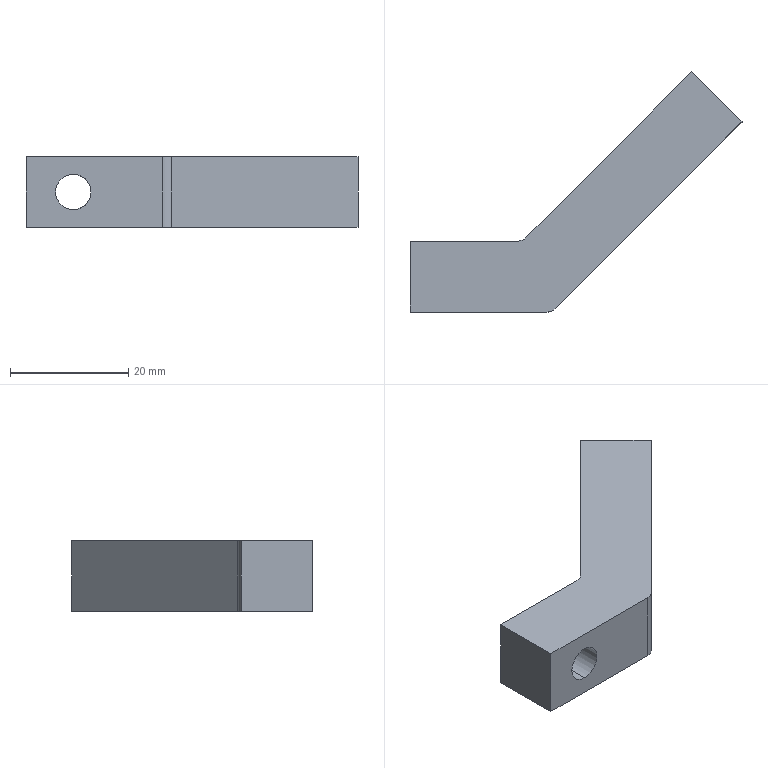CAM job | Mastercam | mm | 14 operations | part box 56.17 x 40.66 x 12
1. Facing | 24 - 100 平铣刀
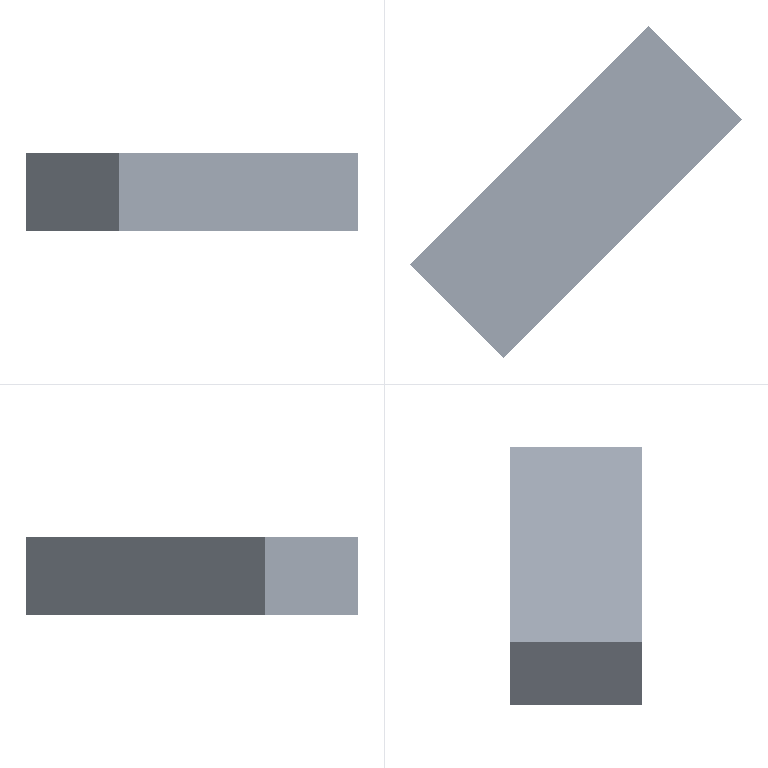2. Contour (Ramp) | 10 - 10 平铣刀
3. Surface Finish Flowline | 11 - 10 圆鼻铣刀
4. Contour (2D) | 10 - 10 平铣刀
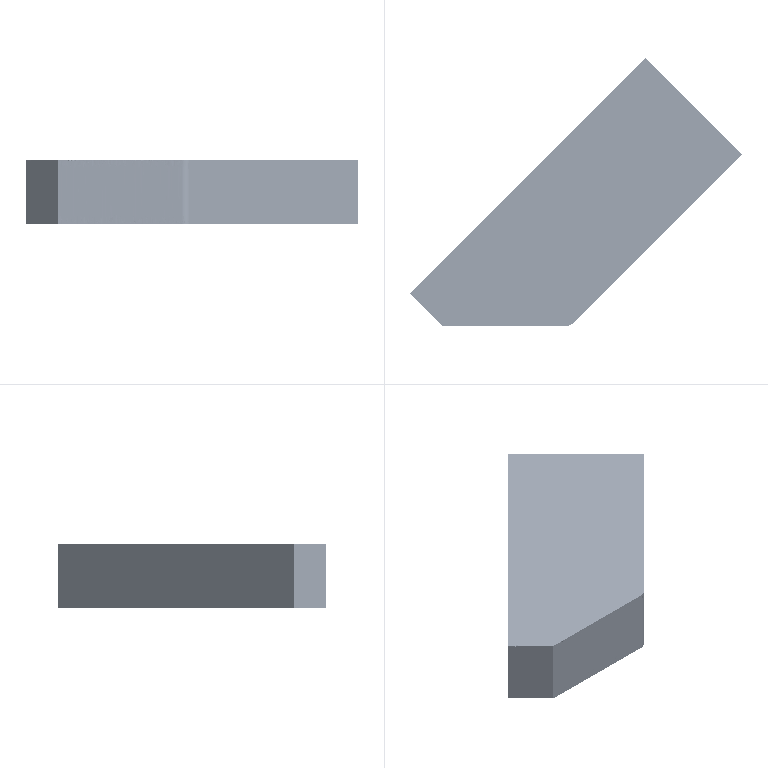5. Deburr 5-axis | 5 - 4 球刀/圆鼻铣刀
6. Facing | 24 - 100 平铣刀
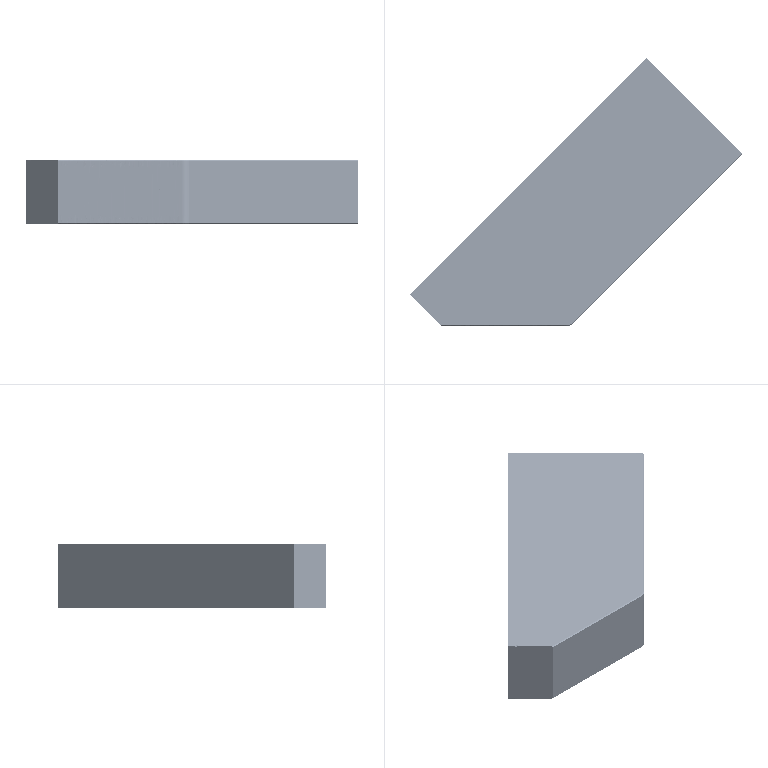7. Contour (2D chamfer) | 7 - 4 倒角刀
8. Drill/Counterbore | 7 - 4 倒角刀
9. Peck Drill | 1 - 6.2 钻头
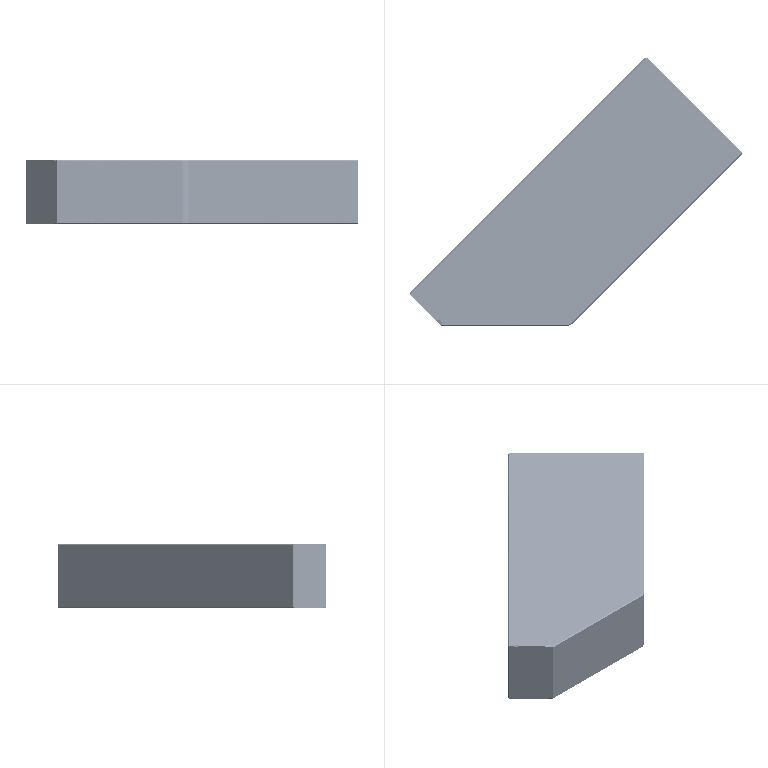10. Contour (Ramp) | 11 - 10 圆鼻铣刀
11. Contour (2D) | 11 - 10 圆鼻铣刀
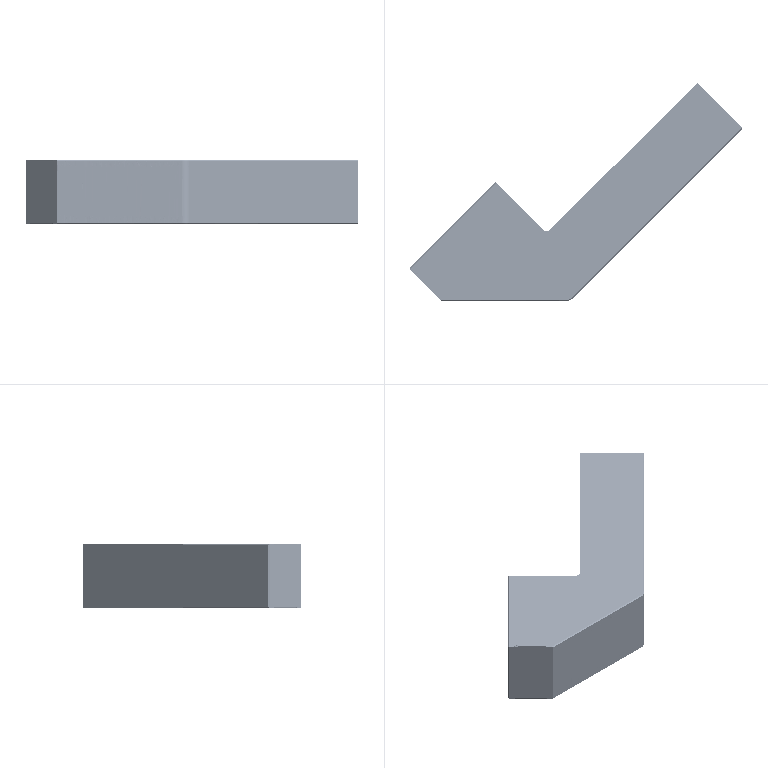12. Surface Finish Flowline | 11 - 10 圆鼻铣刀
13. Deburr 5-axis | 5 - 4 球刀/圆鼻铣刀
14. Drill/Counterbore | 7 - 4 倒角刀